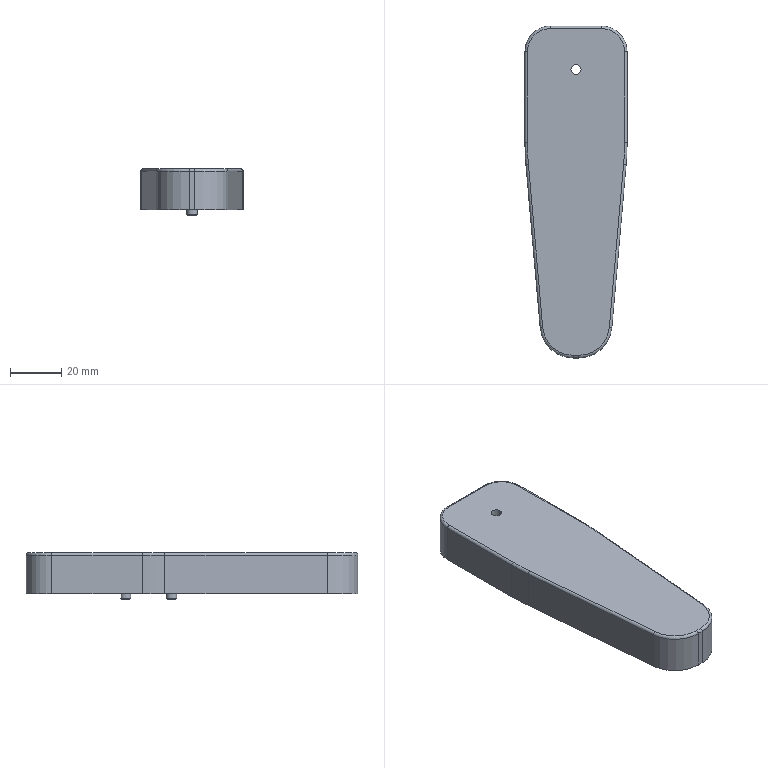Component | NX | CASING | 1 solid | 96 faces | volume 21059 mm3 | cylinder 53 | plane 35 | torus 6 | cone 2 | commonest cylinder face diameters 3 x18 2 x6 6.5 x6 196 x4 6 x3 4 x3 22 x2 16 x2